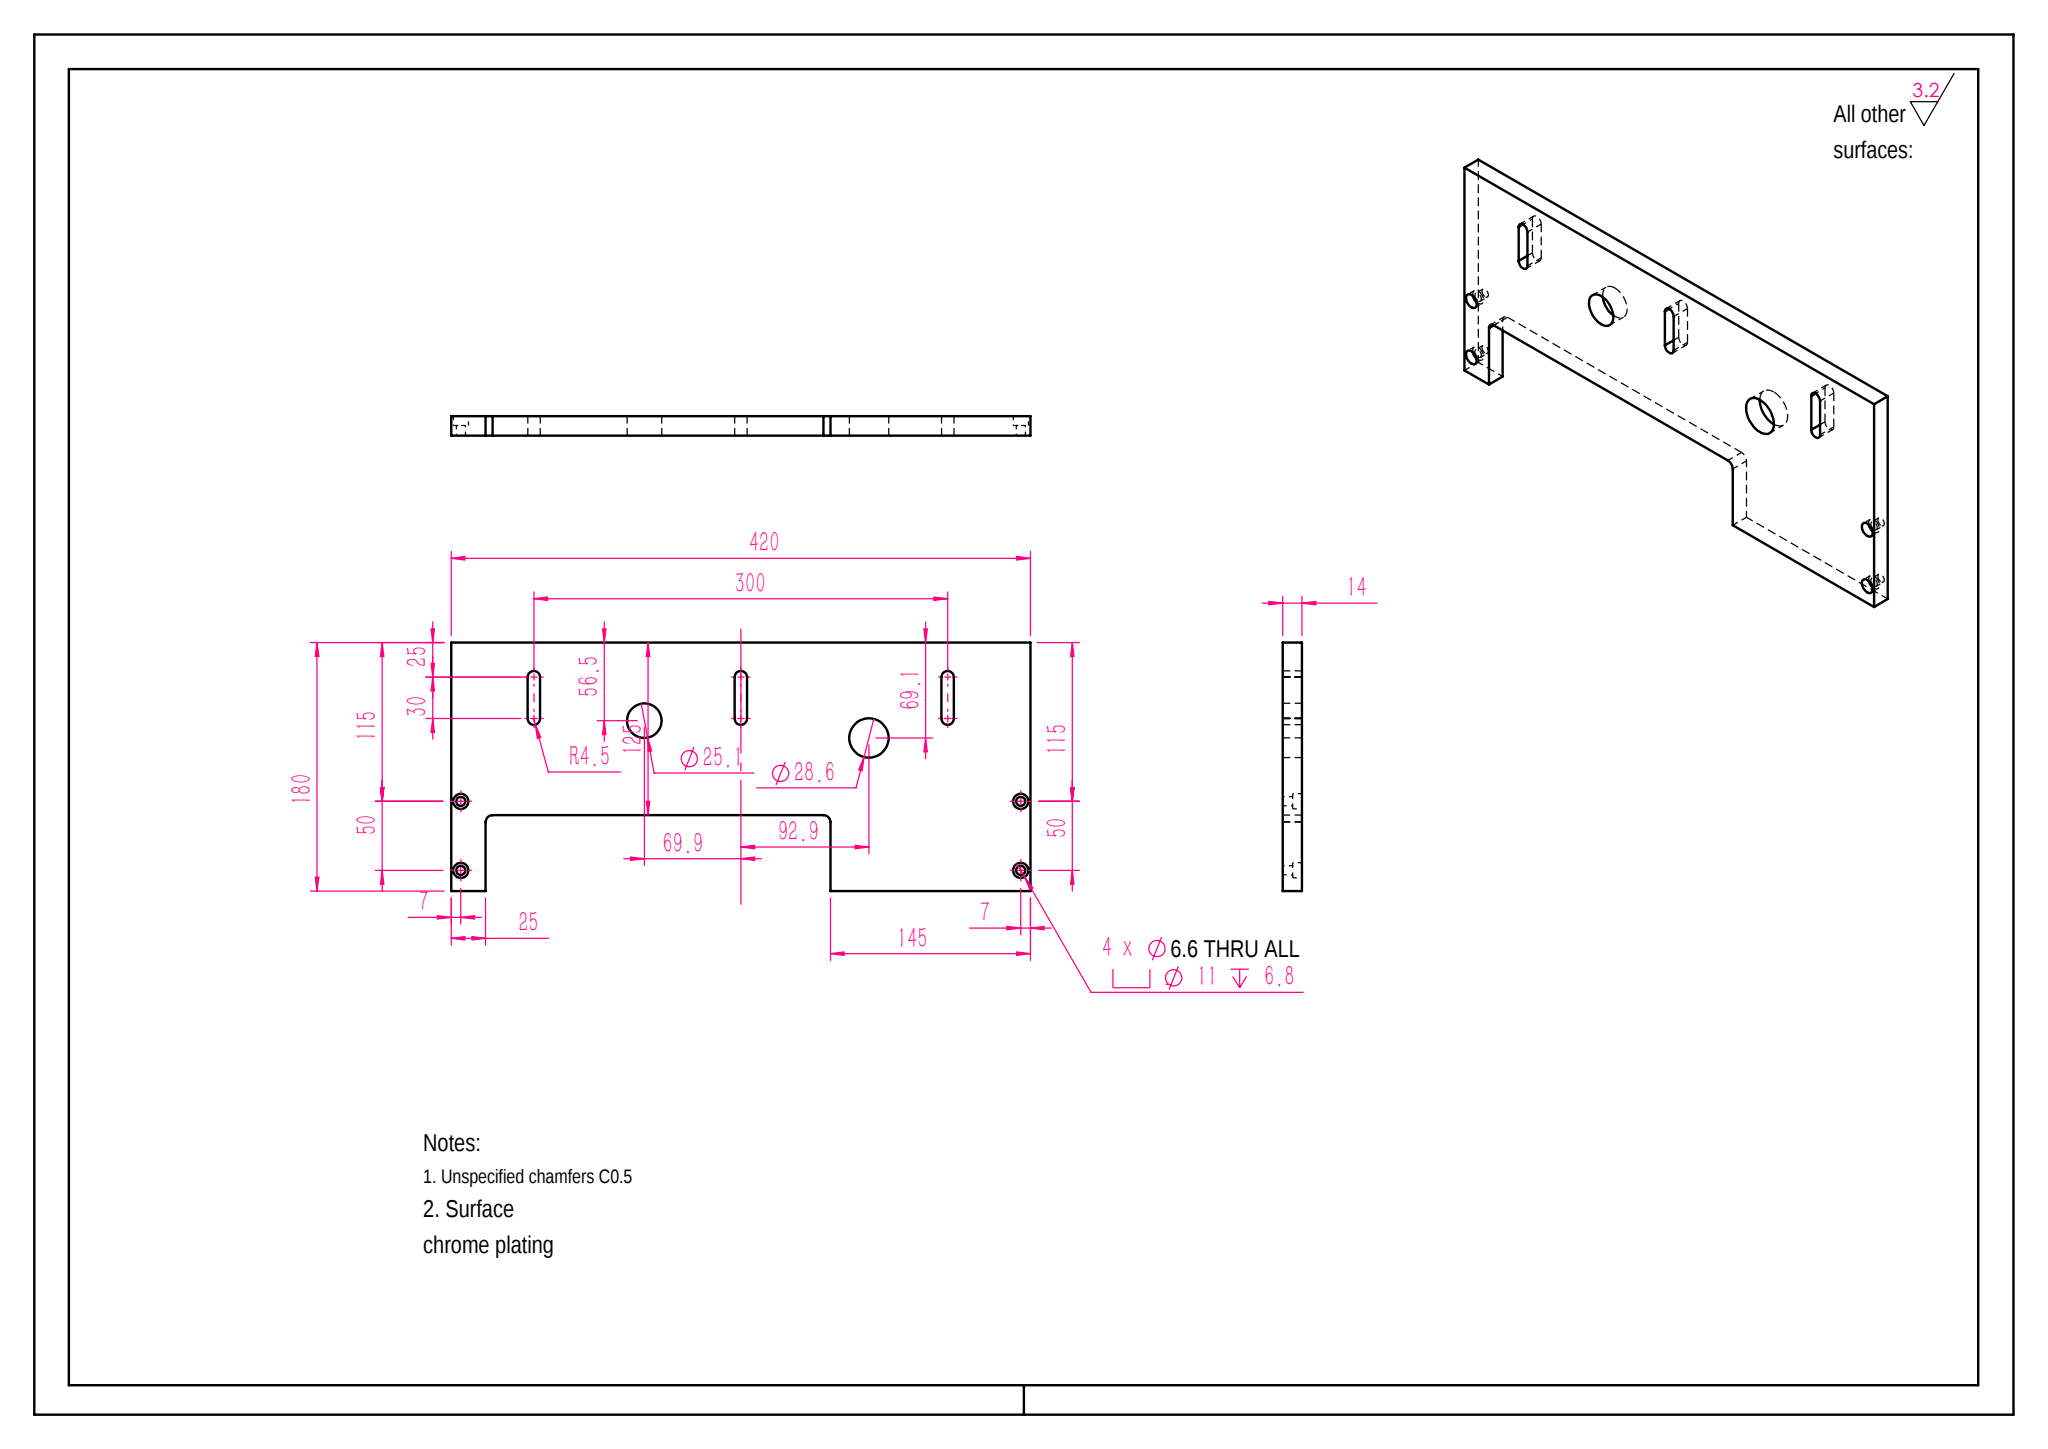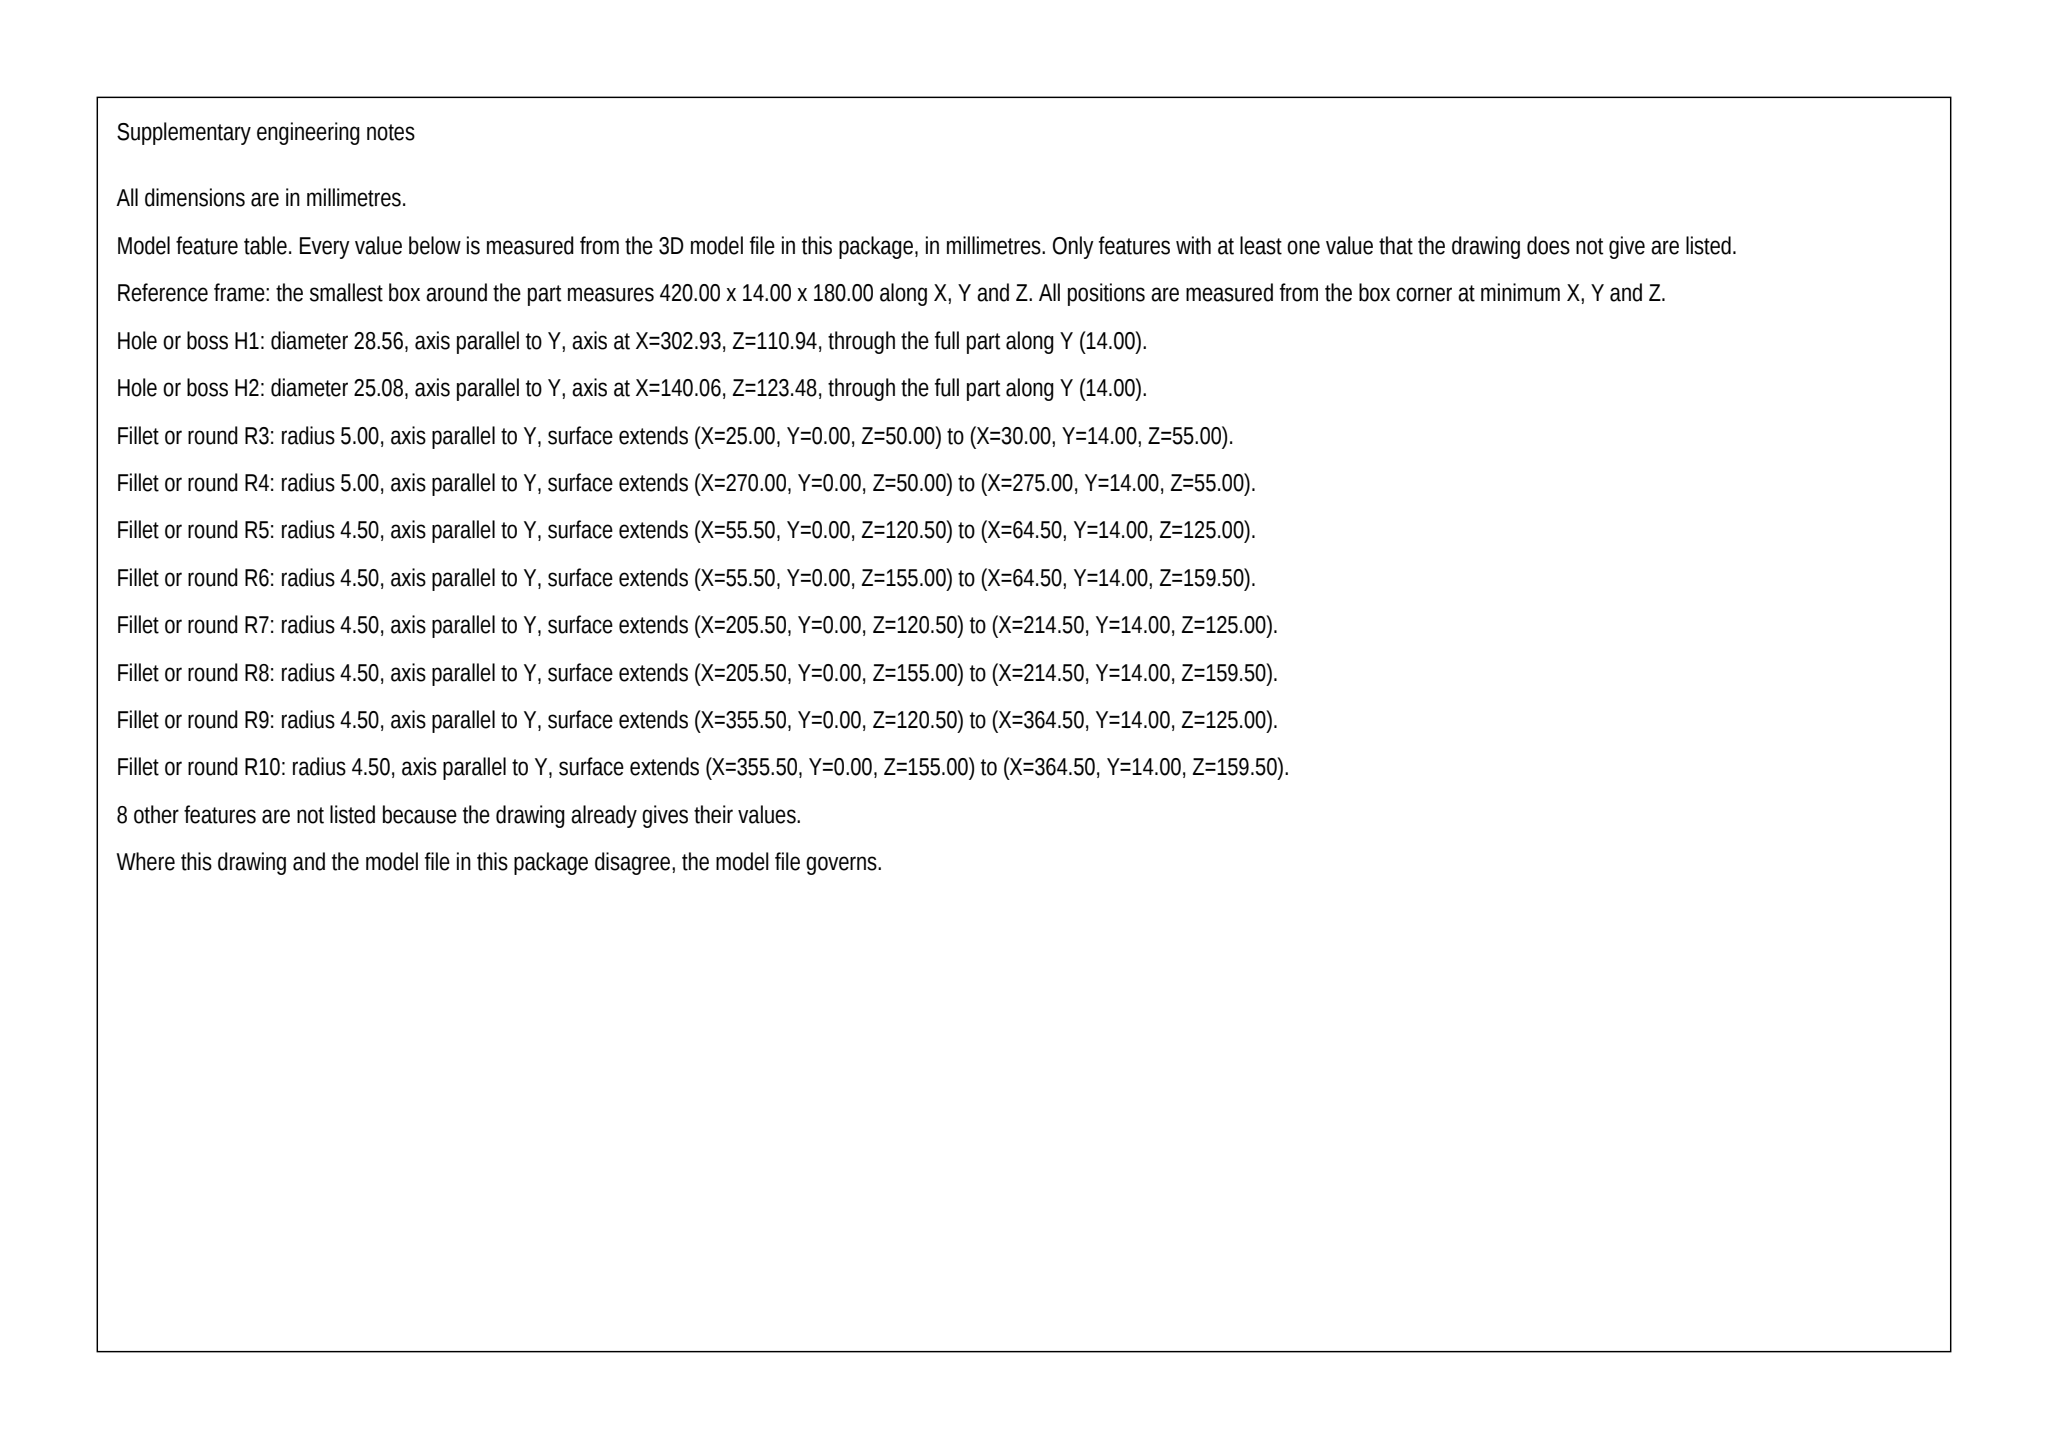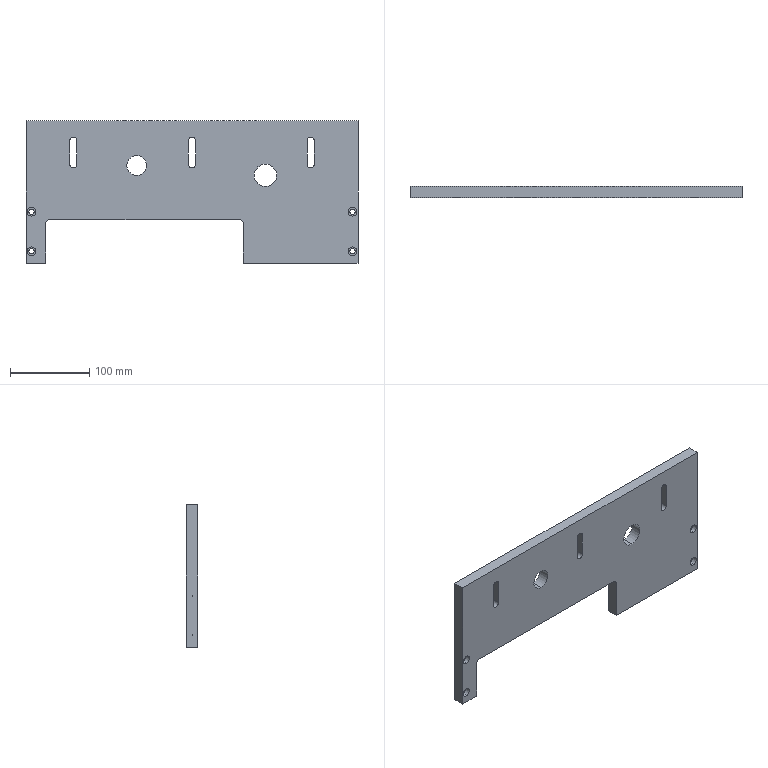Part | SolidWorks | mm | 1 solid | 51 faces | box 420 x 14 x 180 mm | volume 832585 mm3 | cylinder 31 | plane 20 | commonest cylinder face diameters 9 x9 11 x8 6.6 x8 25.075 x2 28.562 x2 10 x2
build123d program:
from build123d import *

# Parameters (mm, degrees)
SKETCH1_W                                            = 420
SKETCH1_H                                            = 180
BOSS_EXTRUDE1_DEPTH                                  = 14
HOLE_SIZE_ACCORDING_TO_HEXAGON_SOCKET_HE_D           = 6.6
HOLE_SIZE_ACCORDING_TO_HEXAGON_SOCKET_HE_CBORE_D     = 11
HOLE_SIZE_ACCORDING_TO_HEXAGON_SOCKET_HE_CBORE_DEPTH = 6.8
CUT_EXTRUDE1_REACH                                   = 230.902
CUT_EXTRUDE2_REACH                                   = 230.902
SKETCH6_R                                            = 12.538
SKETCH6_R_2                                          = 14.281
CUT_EXTRUDE3_DEPTH                                   = 80


with BuildPart() as part:
    # Sketch1 → Boss-Extrude1 (new body)
    with BuildSketch(Plane(origin=(0, 0, 0), x_dir=(1, 0, 0), z_dir=(0, 1, 0))):
        Rectangle(SKETCH1_W, SKETCH1_H)
    extrude(amount=BOSS_EXTRUDE1_DEPTH)

    # Hole Size according to Hexagon Socket He (through all)
    with Locations(Plane(origin=(0, 0, 0), x_dir=(-1, 0, 0), z_dir=(0, -1, 0))):
        with Locations((203, 25), (203, 75), (-203, 25), (-203, 75)):
            CounterBoreHole(HOLE_SIZE_ACCORDING_TO_HEXAGON_SOCKET_HE_D / 2, HOLE_SIZE_ACCORDING_TO_HEXAGON_SOCKET_HE_CBORE_D / 2, HOLE_SIZE_ACCORDING_TO_HEXAGON_SOCKET_HE_CBORE_DEPTH)

    # Sketch4 → Cut-Extrude1 (cut, up to next)
    with BuildSketch(Plane(origin=(0, 14, 0), x_dir=(1, 0, 0), z_dir=(0, 1, 0)), mode=Mode.PRIVATE) as cut_extrude1_sk1:
        with BuildLine():
            Line((-4.5, -65), (-4.5, -35))
            ThreePointArc((-4.5, -35), (0, -30.5), (4.5, -35))
            Line((4.5, -35), (4.5, -65))
            ThreePointArc((4.5, -65), (0, -69.5), (-4.5, -65))
        make_face()
    cut_extrude1_tool1 = extrude(cut_extrude1_sk1.sketch, amount=-CUT_EXTRUDE1_REACH, mode=Mode.PRIVATE) & part.part
    # Sketch4 → Cut-Extrude1 (cut, up to next)
    with BuildSketch(Plane(origin=(0, 14, 0), x_dir=(1, 0, 0), z_dir=(0, 1, 0)), mode=Mode.PRIVATE) as cut_extrude1_sk2:
        with BuildLine():
            Line((-154.5, -65), (-154.5, -35))
            ThreePointArc((-154.5, -35), (-150, -30.5), (-145.5, -35))
            Line((-145.5, -35), (-145.5, -65))
            ThreePointArc((-145.5, -65), (-150, -69.5), (-154.5, -65))
        make_face()
    cut_extrude1_tool2 = extrude(cut_extrude1_sk2.sketch, amount=-CUT_EXTRUDE1_REACH, mode=Mode.PRIVATE) & part.part
    # Sketch4 → Cut-Extrude1 (cut, up to next)
    with BuildSketch(Plane(origin=(0, 14, 0), x_dir=(1, 0, 0), z_dir=(0, 1, 0)), mode=Mode.PRIVATE) as cut_extrude1_sk3:
        with BuildLine():
            Line((145.5, -65), (145.5, -35))
            ThreePointArc((145.5, -35), (150, -30.5), (154.5, -35))
            Line((154.5, -35), (154.5, -65))
            ThreePointArc((154.5, -65), (150, -69.5), (145.5, -65))
        make_face()
    cut_extrude1_tool3 = extrude(cut_extrude1_sk3.sketch, amount=-CUT_EXTRUDE1_REACH, mode=Mode.PRIVATE) & part.part
    add(cut_extrude1_tool1.solids().sort_by_distance((0, 14, 50))[0], mode=Mode.SUBTRACT)
    add(cut_extrude1_tool2.solids().sort_by_distance((-150, 14, 50))[0], mode=Mode.SUBTRACT)
    add(cut_extrude1_tool3.solids().sort_by_distance((150, 14, 50))[0], mode=Mode.SUBTRACT)

    # Sketch5 → Cut-Extrude2 (cut, up to next)
    with BuildSketch(Plane(origin=(0, 14, 0), x_dir=(1, 0, 0), z_dir=(0, 1, 0)), mode=Mode.PRIVATE) as cut_extrude2_sk1:
        with BuildLine():
            Line((65, 90), (-185, 90))
            Line((-185, 90), (-185, 40))
            ThreePointArc((-185, 40), (-183.536, 36.464), (-180, 35))
            Line((-180, 35), (60, 35))
            ThreePointArc((60, 35), (63.536, 36.464), (65, 40))
            Line((65, 40), (65, 90))
        make_face()
    cut_extrude2_tool1 = extrude(cut_extrude2_sk1.sketch, amount=-CUT_EXTRUDE2_REACH, mode=Mode.PRIVATE) & part.part
    add(cut_extrude2_tool1.solids().sort_by_distance((-60, 14, -62.521))[0], mode=Mode.SUBTRACT)

    # Sketch6 → Cut-Extrude3 (cut)
    with BuildSketch(Plane(origin=(0, 14, 0), x_dir=(1, 0, 0), z_dir=(0, 1, 0))):
        with Locations(Location((-69.94, -33.479, 0), (0, 0, 270))):
            Circle(SKETCH6_R)
        with Locations(Location((92.934, -20.941, 0), (0, 0, 270))):
            Circle(SKETCH6_R_2)
    extrude(amount=-CUT_EXTRUDE3_DEPTH, mode=Mode.SUBTRACT)


solid = part.part